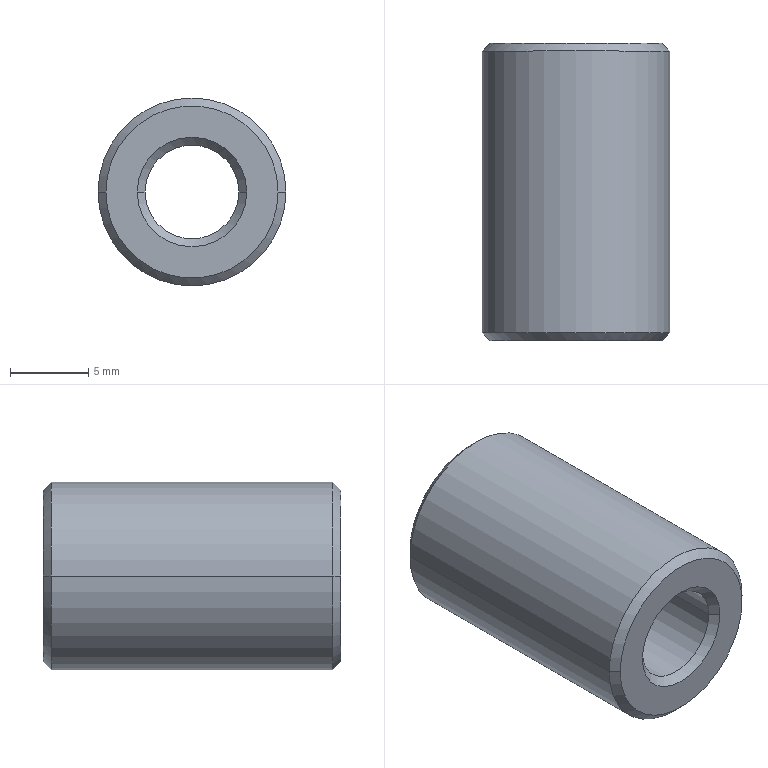Component | SolidWorks | GluePaperFeedingTensioningWheelAssembly-1_YX-04-115GluePaperFeedingTensioningWheelGuideSleeve-1 | 1 solid | 14 faces | box 12 x 19 x 12 mm | volume 1597 mm3 | cone 8 | cylinder 4 | plane 2 | commonest cylinder face diameters 12 x2 6 x2 | material Brass
build123d program:
from build123d import *


with BuildPart() as part:
    # Sketch1 → Revolve1 (revolve)
    with BuildSketch(Plane.XY, mode=Mode.PRIVATE) as revolve1_sk:
        Polygon((-9.5, 3.5), (-9, 3), (9, 3), (9.5, 3.5), (9.5, 5.5), (9, 6), (-9, 6), (-9.5, 5.5), align=None)
    revolve(revolve1_sk.sketch.rotate(Axis((-9.5, 0, 0), (1, 0, 0)), 270), axis=Axis((-9.5, 0, 0), (1, 0, 0)))


solid = part.part

# Placed as in the assembly
solid = solid.moved(Location((29.103, 16.762, 167), (0, 0, 90)))
STEP:
#1=COLOUR_RGB('',0.7922,0.8196,0.9333);
#2=FILL_AREA_STYLE_COLOUR('',#1);
#3=FILL_AREA_STYLE('',(#2));
#4=SURFACE_STYLE_FILL_AREA(#3);
#5=SURFACE_SIDE_STYLE('',(#4));
#6=SURFACE_STYLE_USAGE(.BOTH.,#5);
#7=PRESENTATION_STYLE_ASSIGNMENT((#6));
#8=CARTESIAN_POINT('',(0.9292,1.034,6.575));
#9=VERTEX_POINT('',#8);
#10=CARTESIAN_POINT('',(1.362,1.034,6.575));
#11=VERTEX_POINT('',#10);
#12=CARTESIAN_POINT('',(1.146,1.034,6.575));
#13=DIRECTION('',(0.,-1.,-0.));
#14=DIRECTION('',(-1.,0.,0.));
#15=AXIS2_PLACEMENT_3D('',#12,#13,#14);
#16=CIRCLE('',#15,0.2165);
#17=EDGE_CURVE('',#9,#11,#16,.T.);
#18=ORIENTED_EDGE('',*,*,#17,.T.);
#19=CARTESIAN_POINT('',(1.382,1.014,6.575));
#20=VERTEX_POINT('',#19);
#21=CARTESIAN_POINT('',(1.382,1.014,6.575));
#22=DIRECTION('',(0.7071,-0.7071,-0.));
#23=VECTOR('',#22,39.37);
#24=LINE('',#21,#23);
#25=EDGE_CURVE('',#11,#20,#24,.T.);
#26=ORIENTED_EDGE('',*,*,#25,.T.);
#27=CARTESIAN_POINT('',(0.9096,1.014,6.575));
#28=VERTEX_POINT('',#27);
#29=CARTESIAN_POINT('',(1.146,1.014,6.575));
#30=DIRECTION('',(0.,-1.,-0.));
#31=DIRECTION('',(-1.,0.,0.));
#32=AXIS2_PLACEMENT_3D('',#29,#30,#31);
#33=CIRCLE('',#32,0.2362);
#34=EDGE_CURVE('',#28,#20,#33,.T.);
#35=ORIENTED_EDGE('',*,*,#34,.F.);
#36=CARTESIAN_POINT('',(0.9096,1.014,6.575));
#37=DIRECTION('',(-0.7071,-0.7071,-0.));
#38=VECTOR('',#37,39.37);
#39=LINE('',#36,#38);
#40=EDGE_CURVE('',#9,#28,#39,.T.);
#41=ORIENTED_EDGE('',*,*,#40,.F.);
#42=EDGE_LOOP('',(#18,#26,#35,#41));
#43=FACE_OUTER_BOUND('',#42,.T.);
#44=CARTESIAN_POINT('',(1.146,1.014,6.575));
#45=DIRECTION('',(0.,-1.,-0.));
#46=DIRECTION('',(-1.,0.,0.));
#47=AXIS2_PLACEMENT_3D('',#44,#45,#46);
#48=CONICAL_SURFACE('',#47,0.2362,0.7854);
#49=ADVANCED_FACE('',(#43),#48,.T.);
#50=ORIENTED_EDGE('',*,*,#34,.T.);
#51=CARTESIAN_POINT('',(1.382,0.3056,6.575));
#52=VERTEX_POINT('',#51);
#53=CARTESIAN_POINT('',(1.382,1.034,6.575));
#54=DIRECTION('',(0.,-1.,-0.));
#55=VECTOR('',#54,39.37);
#56=LINE('',#53,#55);
#57=EDGE_CURVE('',#20,#52,#56,.T.);
#58=ORIENTED_EDGE('',*,*,#57,.T.);
#59=CARTESIAN_POINT('',(0.9096,0.3056,6.575));
#60=VERTEX_POINT('',#59);
#61=CARTESIAN_POINT('',(1.146,0.3056,6.575));
#62=DIRECTION('',(0.,-1.,-0.));
#63=DIRECTION('',(-1.,0.,0.));
#64=AXIS2_PLACEMENT_3D('',#61,#62,#63);
#65=CIRCLE('',#64,0.2362);
#66=EDGE_CURVE('',#60,#52,#65,.T.);
#67=ORIENTED_EDGE('',*,*,#66,.F.);
#68=CARTESIAN_POINT('',(0.9096,1.034,6.575));
#69=DIRECTION('',(0.,-1.,-0.));
#70=VECTOR('',#69,39.37);
#71=LINE('',#68,#70);
#72=EDGE_CURVE('',#28,#60,#71,.T.);
#73=ORIENTED_EDGE('',*,*,#72,.F.);
#74=EDGE_LOOP('',(#50,#58,#67,#73));
#75=FACE_OUTER_BOUND('',#74,.T.);
#76=CARTESIAN_POINT('',(1.146,1.034,6.575));
#77=DIRECTION('',(0.,-1.,-0.));
#78=DIRECTION('',(-1.,0.,0.));
#79=AXIS2_PLACEMENT_3D('',#76,#77,#78);
#80=CYLINDRICAL_SURFACE('',#79,0.2362);
#81=ADVANCED_FACE('',(#75),#80,.T.);
#82=CARTESIAN_POINT('',(0.9292,0.2859,6.575));
#83=VERTEX_POINT('',#82);
#84=CARTESIAN_POINT('',(1.362,0.2859,6.575));
#85=VERTEX_POINT('',#84);
#86=CARTESIAN_POINT('',(1.146,0.2859,6.575));
#87=DIRECTION('',(0.,-1.,-0.));
#88=DIRECTION('',(-1.,0.,0.));
#89=AXIS2_PLACEMENT_3D('',#86,#87,#88);
#90=CIRCLE('',#89,0.2165);
#91=EDGE_CURVE('',#83,#85,#90,.T.);
#92=ORIENTED_EDGE('',*,*,#91,.F.);
#93=CARTESIAN_POINT('',(0.9292,0.2859,6.575));
#94=DIRECTION('',(-0.7071,0.7071,-0.));
#95=VECTOR('',#94,39.37);
#96=LINE('',#93,#95);
#97=EDGE_CURVE('',#83,#60,#96,.T.);
#98=ORIENTED_EDGE('',*,*,#97,.T.);
#99=ORIENTED_EDGE('',*,*,#66,.T.);
#100=CARTESIAN_POINT('',(1.362,0.2859,6.575));
#101=DIRECTION('',(0.7071,0.7071,0.));
#102=VECTOR('',#101,39.37);
#103=LINE('',#100,#102);
#104=EDGE_CURVE('',#85,#52,#103,.T.);
#105=ORIENTED_EDGE('',*,*,#104,.F.);
#106=EDGE_LOOP('',(#92,#98,#99,#105));
#107=FACE_OUTER_BOUND('',#106,.T.);
#108=CARTESIAN_POINT('',(1.146,0.2859,6.575));
#109=DIRECTION('',(-0.,1.,0.));
#110=DIRECTION('',(1.,0.,0.));
#111=AXIS2_PLACEMENT_3D('',#108,#109,#110);
#112=CONICAL_SURFACE('',#111,0.2165,0.7854);
#113=ADVANCED_FACE('',(#107),#112,.T.);
#114=CARTESIAN_POINT('',(1.264,0.3056,6.575));
#115=VERTEX_POINT('',#114);
#116=CARTESIAN_POINT('',(1.028,0.3056,6.575));
#117=VERTEX_POINT('',#116);
#118=CARTESIAN_POINT('',(1.146,0.3056,6.575));
#119=DIRECTION('',(0.,-1.,-0.));
#120=DIRECTION('',(-1.,0.,0.));
#121=AXIS2_PLACEMENT_3D('',#118,#119,#120);
#122=CIRCLE('',#121,0.1181);
#123=EDGE_CURVE('',#115,#117,#122,.T.);
#124=ORIENTED_EDGE('',*,*,#123,.F.);
#125=CARTESIAN_POINT('',(1.284,0.2859,6.575));
#126=VERTEX_POINT('',#125);
#127=CARTESIAN_POINT('',(1.264,0.3056,6.575));
#128=DIRECTION('',(0.7071,-0.7071,-0.));
#129=VECTOR('',#128,39.37);
#130=LINE('',#127,#129);
#131=EDGE_CURVE('',#115,#126,#130,.T.);
#132=ORIENTED_EDGE('',*,*,#131,.T.);
#133=CARTESIAN_POINT('',(1.008,0.2859,6.575));
#134=VERTEX_POINT('',#133);
#135=CARTESIAN_POINT('',(1.146,0.2859,6.575));
#136=DIRECTION('',(0.,-1.,-0.));
#137=DIRECTION('',(-1.,0.,0.));
#138=AXIS2_PLACEMENT_3D('',#135,#136,#137);
#139=CIRCLE('',#138,0.1378);
#140=EDGE_CURVE('',#126,#134,#139,.T.);
#141=ORIENTED_EDGE('',*,*,#140,.T.);
#142=CARTESIAN_POINT('',(1.028,0.3056,6.575));
#143=DIRECTION('',(-0.7071,-0.7071,-0.));
#144=VECTOR('',#143,39.37);
#145=LINE('',#142,#144);
#146=EDGE_CURVE('',#117,#134,#145,.T.);
#147=ORIENTED_EDGE('',*,*,#146,.F.);
#148=EDGE_LOOP('',(#124,#132,#141,#147));
#149=FACE_OUTER_BOUND('',#148,.T.);
#150=CARTESIAN_POINT('',(1.146,0.3056,6.575));
#151=DIRECTION('',(0.,-1.,-0.));
#152=DIRECTION('',(-1.,0.,0.));
#153=AXIS2_PLACEMENT_3D('',#150,#151,#152);
#154=CONICAL_SURFACE('',#153,0.1181,0.7854);
#155=ADVANCED_FACE('',(#149),#154,.F.);
#156=CARTESIAN_POINT('',(1.264,1.014,6.575));
#157=VERTEX_POINT('',#156);
#158=CARTESIAN_POINT('',(1.028,1.014,6.575));
#159=VERTEX_POINT('',#158);
#160=CARTESIAN_POINT('',(1.146,1.014,6.575));
#161=DIRECTION('',(0.,-1.,-0.));
#162=DIRECTION('',(-1.,0.,0.));
#163=AXIS2_PLACEMENT_3D('',#160,#161,#162);
#164=CIRCLE('',#163,0.1181);
#165=EDGE_CURVE('',#157,#159,#164,.T.);
#166=ORIENTED_EDGE('',*,*,#165,.F.);
#167=CARTESIAN_POINT('',(1.264,1.034,6.575));
#168=DIRECTION('',(0.,-1.,-0.));
#169=VECTOR('',#168,39.37);
#170=LINE('',#167,#169);
#171=EDGE_CURVE('',#157,#115,#170,.T.);
#172=ORIENTED_EDGE('',*,*,#171,.T.);
#173=ORIENTED_EDGE('',*,*,#123,.T.);
#174=CARTESIAN_POINT('',(1.028,1.034,6.575));
#175=DIRECTION('',(0.,-1.,-0.));
#176=VECTOR('',#175,39.37);
#177=LINE('',#174,#176);
#178=EDGE_CURVE('',#159,#117,#177,.T.);
#179=ORIENTED_EDGE('',*,*,#178,.F.);
#180=EDGE_LOOP('',(#166,#172,#173,#179));
#181=FACE_OUTER_BOUND('',#180,.T.);
#182=CARTESIAN_POINT('',(1.146,1.034,6.575));
#183=DIRECTION('',(0.,-1.,-0.));
#184=DIRECTION('',(-1.,0.,0.));
#185=AXIS2_PLACEMENT_3D('',#182,#183,#184);
#186=CYLINDRICAL_SURFACE('',#185,0.1181);
#187=ADVANCED_FACE('',(#181),#186,.F.);
#188=ORIENTED_EDGE('',*,*,#165,.T.);
#189=CARTESIAN_POINT('',(1.008,1.034,6.575));
#190=VERTEX_POINT('',#189);
#191=CARTESIAN_POINT('',(1.008,1.034,6.575));
#192=DIRECTION('',(-0.7071,0.7071,-0.));
#193=VECTOR('',#192,39.37);
#194=LINE('',#191,#193);
#195=EDGE_CURVE('',#159,#190,#194,.T.);
#196=ORIENTED_EDGE('',*,*,#195,.T.);
#197=CARTESIAN_POINT('',(1.284,1.034,6.575));
#198=VERTEX_POINT('',#197);
#199=CARTESIAN_POINT('',(1.146,1.034,6.575));
#200=DIRECTION('',(0.,-1.,-0.));
#201=DIRECTION('',(-1.,0.,0.));
#202=AXIS2_PLACEMENT_3D('',#199,#200,#201);
#203=CIRCLE('',#202,0.1378);
#204=EDGE_CURVE('',#198,#190,#203,.T.);
#205=ORIENTED_EDGE('',*,*,#204,.F.);
#206=CARTESIAN_POINT('',(1.284,1.034,6.575));
#207=DIRECTION('',(0.7071,0.7071,0.));
#208=VECTOR('',#207,39.37);
#209=LINE('',#206,#208);
#210=EDGE_CURVE('',#157,#198,#209,.T.);
#211=ORIENTED_EDGE('',*,*,#210,.F.);
#212=EDGE_LOOP('',(#188,#196,#205,#211));
#213=FACE_OUTER_BOUND('',#212,.T.);
#214=CARTESIAN_POINT('',(1.146,1.034,6.575));
#215=DIRECTION('',(-0.,1.,0.));
#216=DIRECTION('',(1.,0.,0.));
#217=AXIS2_PLACEMENT_3D('',#214,#215,#216);
#218=CONICAL_SURFACE('',#217,0.1378,0.7854);
#219=ADVANCED_FACE('',(#213),#218,.F.);
#220=ORIENTED_EDGE('',*,*,#204,.T.);
#221=CARTESIAN_POINT('',(1.146,1.034,6.575));
#222=DIRECTION('',(0.,-1.,-0.));
#223=DIRECTION('',(-1.,0.,0.));
#224=AXIS2_PLACEMENT_3D('',#221,#222,#223);
#225=CIRCLE('',#224,0.1378);
#226=EDGE_CURVE('',#190,#198,#225,.T.);
#227=ORIENTED_EDGE('',*,*,#226,.T.);
#228=EDGE_LOOP('',(#220,#227));
#229=FACE_BOUND('',#228,.T.);
#230=ORIENTED_EDGE('',*,*,#17,.F.);
#231=CARTESIAN_POINT('',(1.146,1.034,6.575));
#232=DIRECTION('',(0.,-1.,-0.));
#233=DIRECTION('',(-1.,0.,0.));
#234=AXIS2_PLACEMENT_3D('',#231,#232,#233);
#235=CIRCLE('',#234,0.2165);
#236=EDGE_CURVE('',#11,#9,#235,.T.);
#237=ORIENTED_EDGE('',*,*,#236,.F.);
#238=EDGE_LOOP('',(#230,#237));
#239=FACE_OUTER_BOUND('',#238,.T.);
#240=CARTESIAN_POINT('',(1.146,1.034,6.358));
#241=DIRECTION('',(-0.,1.,0.));
#242=DIRECTION('',(1.,0.,0.));
#243=AXIS2_PLACEMENT_3D('',#240,#241,#242);
#244=PLANE('',#243);
#245=ADVANCED_FACE('',(#229,#239),#244,.T.);
#246=ORIENTED_EDGE('',*,*,#195,.F.);
#247=CARTESIAN_POINT('',(1.146,1.014,6.575));
#248=DIRECTION('',(0.,-1.,-0.));
#249=DIRECTION('',(-1.,0.,0.));
#250=AXIS2_PLACEMENT_3D('',#247,#248,#249);
#251=CIRCLE('',#250,0.1181);
#252=EDGE_CURVE('',#159,#157,#251,.T.);
#253=ORIENTED_EDGE('',*,*,#252,.T.);
#254=ORIENTED_EDGE('',*,*,#210,.T.);
#255=ORIENTED_EDGE('',*,*,#226,.F.);
#256=EDGE_LOOP('',(#246,#253,#254,#255));
#257=FACE_OUTER_BOUND('',#256,.T.);
#258=CARTESIAN_POINT('',(1.146,1.034,6.575));
#259=DIRECTION('',(-0.,1.,0.));
#260=DIRECTION('',(1.,0.,0.));
#261=AXIS2_PLACEMENT_3D('',#258,#259,#260);
#262=CONICAL_SURFACE('',#261,0.1378,0.7854);
#263=ADVANCED_FACE('',(#257),#262,.F.);
#264=ORIENTED_EDGE('',*,*,#171,.F.);
#265=ORIENTED_EDGE('',*,*,#252,.F.);
#266=ORIENTED_EDGE('',*,*,#178,.T.);
#267=CARTESIAN_POINT('',(1.146,0.3056,6.575));
#268=DIRECTION('',(0.,-1.,-0.));
#269=DIRECTION('',(-1.,0.,0.));
#270=AXIS2_PLACEMENT_3D('',#267,#268,#269);
#271=CIRCLE('',#270,0.1181);
#272=EDGE_CURVE('',#117,#115,#271,.T.);
#273=ORIENTED_EDGE('',*,*,#272,.T.);
#274=EDGE_LOOP('',(#264,#265,#266,#273));
#275=FACE_OUTER_BOUND('',#274,.T.);
#276=CARTESIAN_POINT('',(1.146,1.034,6.575));
#277=DIRECTION('',(0.,-1.,-0.));
#278=DIRECTION('',(-1.,0.,0.));
#279=AXIS2_PLACEMENT_3D('',#276,#277,#278);
#280=CYLINDRICAL_SURFACE('',#279,0.1181);
#281=ADVANCED_FACE('',(#275),#280,.F.);
#282=ORIENTED_EDGE('',*,*,#131,.F.);
#283=ORIENTED_EDGE('',*,*,#272,.F.);
#284=ORIENTED_EDGE('',*,*,#146,.T.);
#285=CARTESIAN_POINT('',(1.146,0.2859,6.575));
#286=DIRECTION('',(0.,-1.,-0.));
#287=DIRECTION('',(-1.,0.,0.));
#288=AXIS2_PLACEMENT_3D('',#285,#286,#287);
#289=CIRCLE('',#288,0.1378);
#290=EDGE_CURVE('',#134,#126,#289,.T.);
#291=ORIENTED_EDGE('',*,*,#290,.T.);
#292=EDGE_LOOP('',(#282,#283,#284,#291));
#293=FACE_OUTER_BOUND('',#292,.T.);
#294=CARTESIAN_POINT('',(1.146,0.3056,6.575));
#295=DIRECTION('',(0.,-1.,-0.));
#296=DIRECTION('',(-1.,0.,0.));
#297=AXIS2_PLACEMENT_3D('',#294,#295,#296);
#298=CONICAL_SURFACE('',#297,0.1181,0.7854);
#299=ADVANCED_FACE('',(#293),#298,.F.);
#300=CARTESIAN_POINT('',(1.146,0.2859,6.575));
#301=DIRECTION('',(0.,-1.,-0.));
#302=DIRECTION('',(-1.,0.,0.));
#303=AXIS2_PLACEMENT_3D('',#300,#301,#302);
#304=CIRCLE('',#303,0.2165);
#305=EDGE_CURVE('',#85,#83,#304,.T.);
#306=ORIENTED_EDGE('',*,*,#305,.T.);
#307=ORIENTED_EDGE('',*,*,#91,.T.);
#308=EDGE_LOOP('',(#306,#307));
#309=FACE_OUTER_BOUND('',#308,.T.);
#310=ORIENTED_EDGE('',*,*,#290,.F.);
#311=ORIENTED_EDGE('',*,*,#140,.F.);
#312=EDGE_LOOP('',(#310,#311));
#313=FACE_BOUND('',#312,.T.);
#314=CARTESIAN_POINT('',(1.146,0.2859,6.437));
#315=DIRECTION('',(0.,-1.,-0.));
#316=DIRECTION('',(-1.,-0.,-0.));
#317=AXIS2_PLACEMENT_3D('',#314,#315,#316);
#318=PLANE('',#317);
#319=ADVANCED_FACE('',(#309,#313),#318,.T.);
#320=ORIENTED_EDGE('',*,*,#97,.F.);
#321=ORIENTED_EDGE('',*,*,#305,.F.);
#322=ORIENTED_EDGE('',*,*,#104,.T.);
#323=CARTESIAN_POINT('',(1.146,0.3056,6.575));
#324=DIRECTION('',(0.,-1.,-0.));
#325=DIRECTION('',(-1.,0.,0.));
#326=AXIS2_PLACEMENT_3D('',#323,#324,#325);
#327=CIRCLE('',#326,0.2362);
#328=EDGE_CURVE('',#52,#60,#327,.T.);
#329=ORIENTED_EDGE('',*,*,#328,.T.);
#330=EDGE_LOOP('',(#320,#321,#322,#329));
#331=FACE_OUTER_BOUND('',#330,.T.);
#332=CARTESIAN_POINT('',(1.146,0.2859,6.575));
#333=DIRECTION('',(-0.,1.,0.));
#334=DIRECTION('',(1.,0.,0.));
#335=AXIS2_PLACEMENT_3D('',#332,#333,#334);
#336=CONICAL_SURFACE('',#335,0.2165,0.7854);
#337=ADVANCED_FACE('',(#331),#336,.T.);
#338=ORIENTED_EDGE('',*,*,#57,.F.);
#339=CARTESIAN_POINT('',(1.146,1.014,6.575));
#340=DIRECTION('',(0.,-1.,-0.));
#341=DIRECTION('',(-1.,0.,0.));
#342=AXIS2_PLACEMENT_3D('',#339,#340,#341);
#343=CIRCLE('',#342,0.2362);
#344=EDGE_CURVE('',#20,#28,#343,.T.);
#345=ORIENTED_EDGE('',*,*,#344,.T.);
#346=ORIENTED_EDGE('',*,*,#72,.T.);
#347=ORIENTED_EDGE('',*,*,#328,.F.);
#348=EDGE_LOOP('',(#338,#345,#346,#347));
#349=FACE_OUTER_BOUND('',#348,.T.);
#350=CARTESIAN_POINT('',(1.146,1.034,6.575));
#351=DIRECTION('',(0.,-1.,-0.));
#352=DIRECTION('',(-1.,0.,0.));
#353=AXIS2_PLACEMENT_3D('',#350,#351,#352);
#354=CYLINDRICAL_SURFACE('',#353,0.2362);
#355=ADVANCED_FACE('',(#349),#354,.T.);
#356=ORIENTED_EDGE('',*,*,#25,.F.);
#357=ORIENTED_EDGE('',*,*,#236,.T.);
#358=ORIENTED_EDGE('',*,*,#40,.T.);
#359=ORIENTED_EDGE('',*,*,#344,.F.);
#360=EDGE_LOOP('',(#356,#357,#358,#359));
#361=FACE_OUTER_BOUND('',#360,.T.);
#362=CARTESIAN_POINT('',(1.146,1.014,6.575));
#363=DIRECTION('',(0.,-1.,-0.));
#364=DIRECTION('',(-1.,0.,0.));
#365=AXIS2_PLACEMENT_3D('',#362,#363,#364);
#366=CONICAL_SURFACE('',#365,0.2362,0.7854);
#367=ADVANCED_FACE('',(#361),#366,.T.);
#368=CLOSED_SHELL('',(#49,#81,#113,#155,#187,#219,#245,#263,#281,#299,#319,#337,#355,#367));
#369=MANIFOLD_SOLID_BREP('',#368);
#370=STYLED_ITEM('',(#7),#369);
#371=PRESENTATION_LAYER_ASSIGNMENT('','',(#370));
#372=CARTESIAN_POINT('',(0.,0.,0.));
#373=DIRECTION('',(0.,0.,1.));
#374=DIRECTION('',(1.,0.,0.));
#375=AXIS2_PLACEMENT_3D('',#372,#373,#374);
#376=(LENGTH_UNIT()NAMED_UNIT(*)SI_UNIT($,.METRE.));
#377=LENGTH_MEASURE_WITH_UNIT(LENGTH_MEASURE(0.0254),#376);
#378=DIMENSIONAL_EXPONENTS(1.,0.,0.,0.,0.,0.,0.);
#379=(CONVERSION_BASED_UNIT('',#377)LENGTH_UNIT()NAMED_UNIT(#378));
#380=UNCERTAINTY_MEASURE_WITH_UNIT(LENGTH_MEASURE(0.00001),#379,'','');
#381=(NAMED_UNIT(*)PLANE_ANGLE_UNIT()SI_UNIT($,.RADIAN.));
#382=(NAMED_UNIT(*)SI_UNIT($,.STERADIAN.)SOLID_ANGLE_UNIT());
#383=(GEOMETRIC_REPRESENTATION_CONTEXT(3)GLOBAL_UNCERTAINTY_ASSIGNED_CONTEXT((#380))GLOBAL_UNIT_ASSIGNED_CONTEXT((#379,#381,#382))REPRESENTATION_CONTEXT('',''));
#384=ADVANCED_BREP_SHAPE_REPRESENTATION('',(#369,#375),#383);
#385=(LENGTH_UNIT()NAMED_UNIT(*)SI_UNIT($,.METRE.));
#386=LENGTH_MEASURE_WITH_UNIT(LENGTH_MEASURE(0.0254),#385);
#387=DIMENSIONAL_EXPONENTS(1.,0.,0.,0.,0.,0.,0.);
#388=(CONVERSION_BASED_UNIT('',#386)LENGTH_UNIT()NAMED_UNIT(#387));
#389=UNCERTAINTY_MEASURE_WITH_UNIT(LENGTH_MEASURE(0.00001),#388,'','');
#390=(NAMED_UNIT(*)PLANE_ANGLE_UNIT()SI_UNIT($,.RADIAN.));
#391=(NAMED_UNIT(*)SI_UNIT($,.STERADIAN.)SOLID_ANGLE_UNIT());
#392=(GEOMETRIC_REPRESENTATION_CONTEXT(3)GLOBAL_UNCERTAINTY_ASSIGNED_CONTEXT((#389))GLOBAL_UNIT_ASSIGNED_CONTEXT((#388,#390,#391))REPRESENTATION_CONTEXT('',''));
#393=MECHANICAL_DESIGN_GEOMETRIC_PRESENTATION_REPRESENTATION('',(#370),#392);